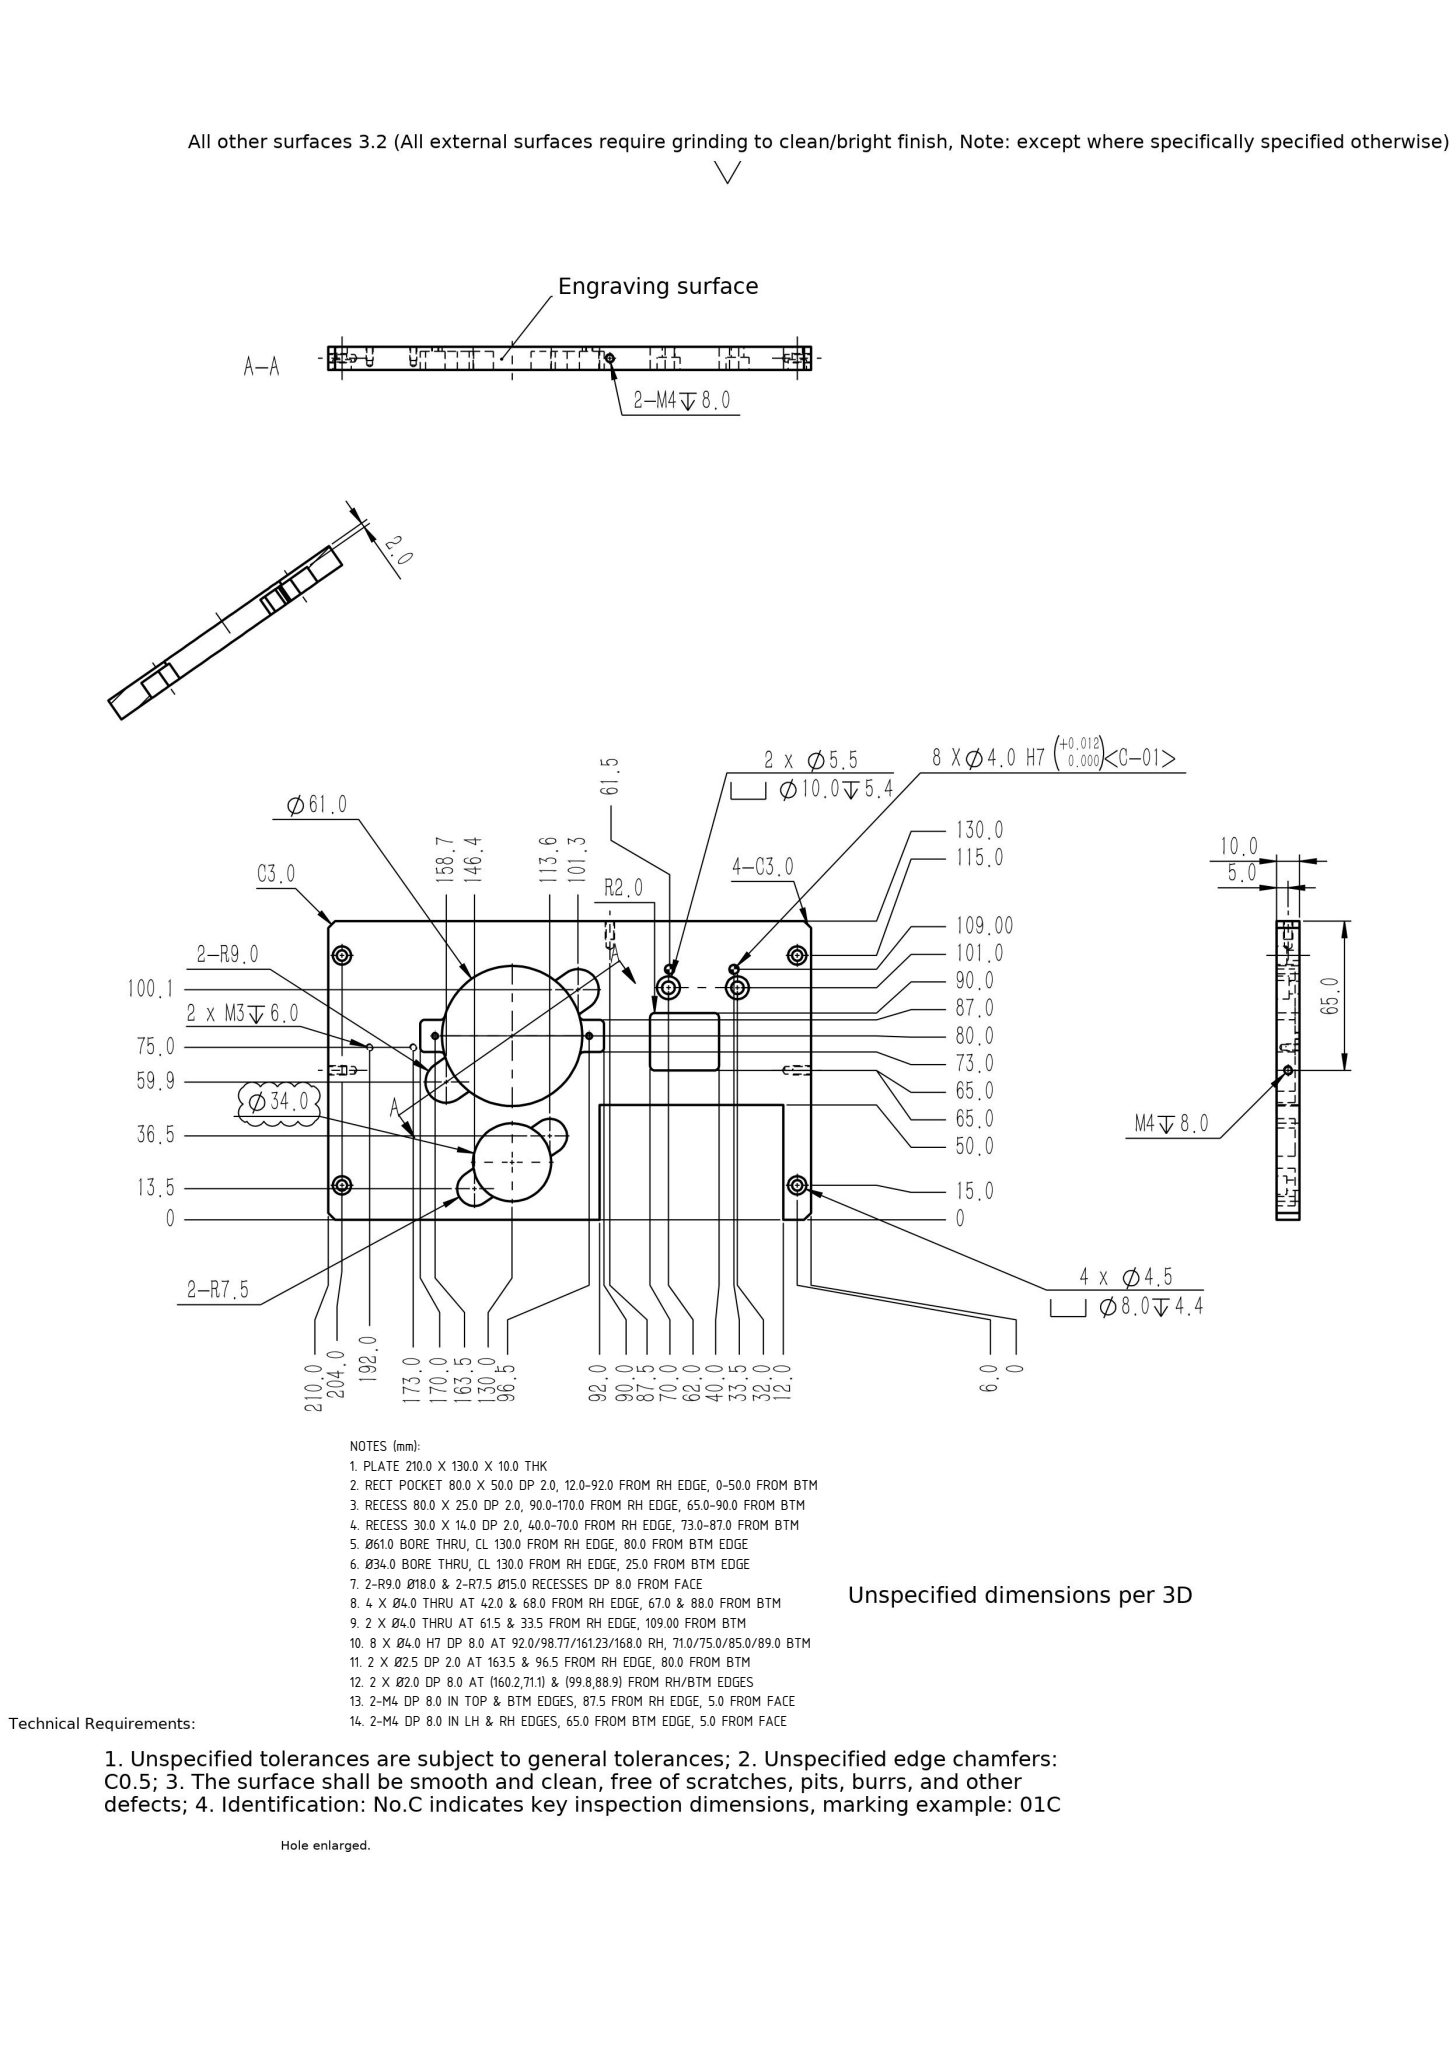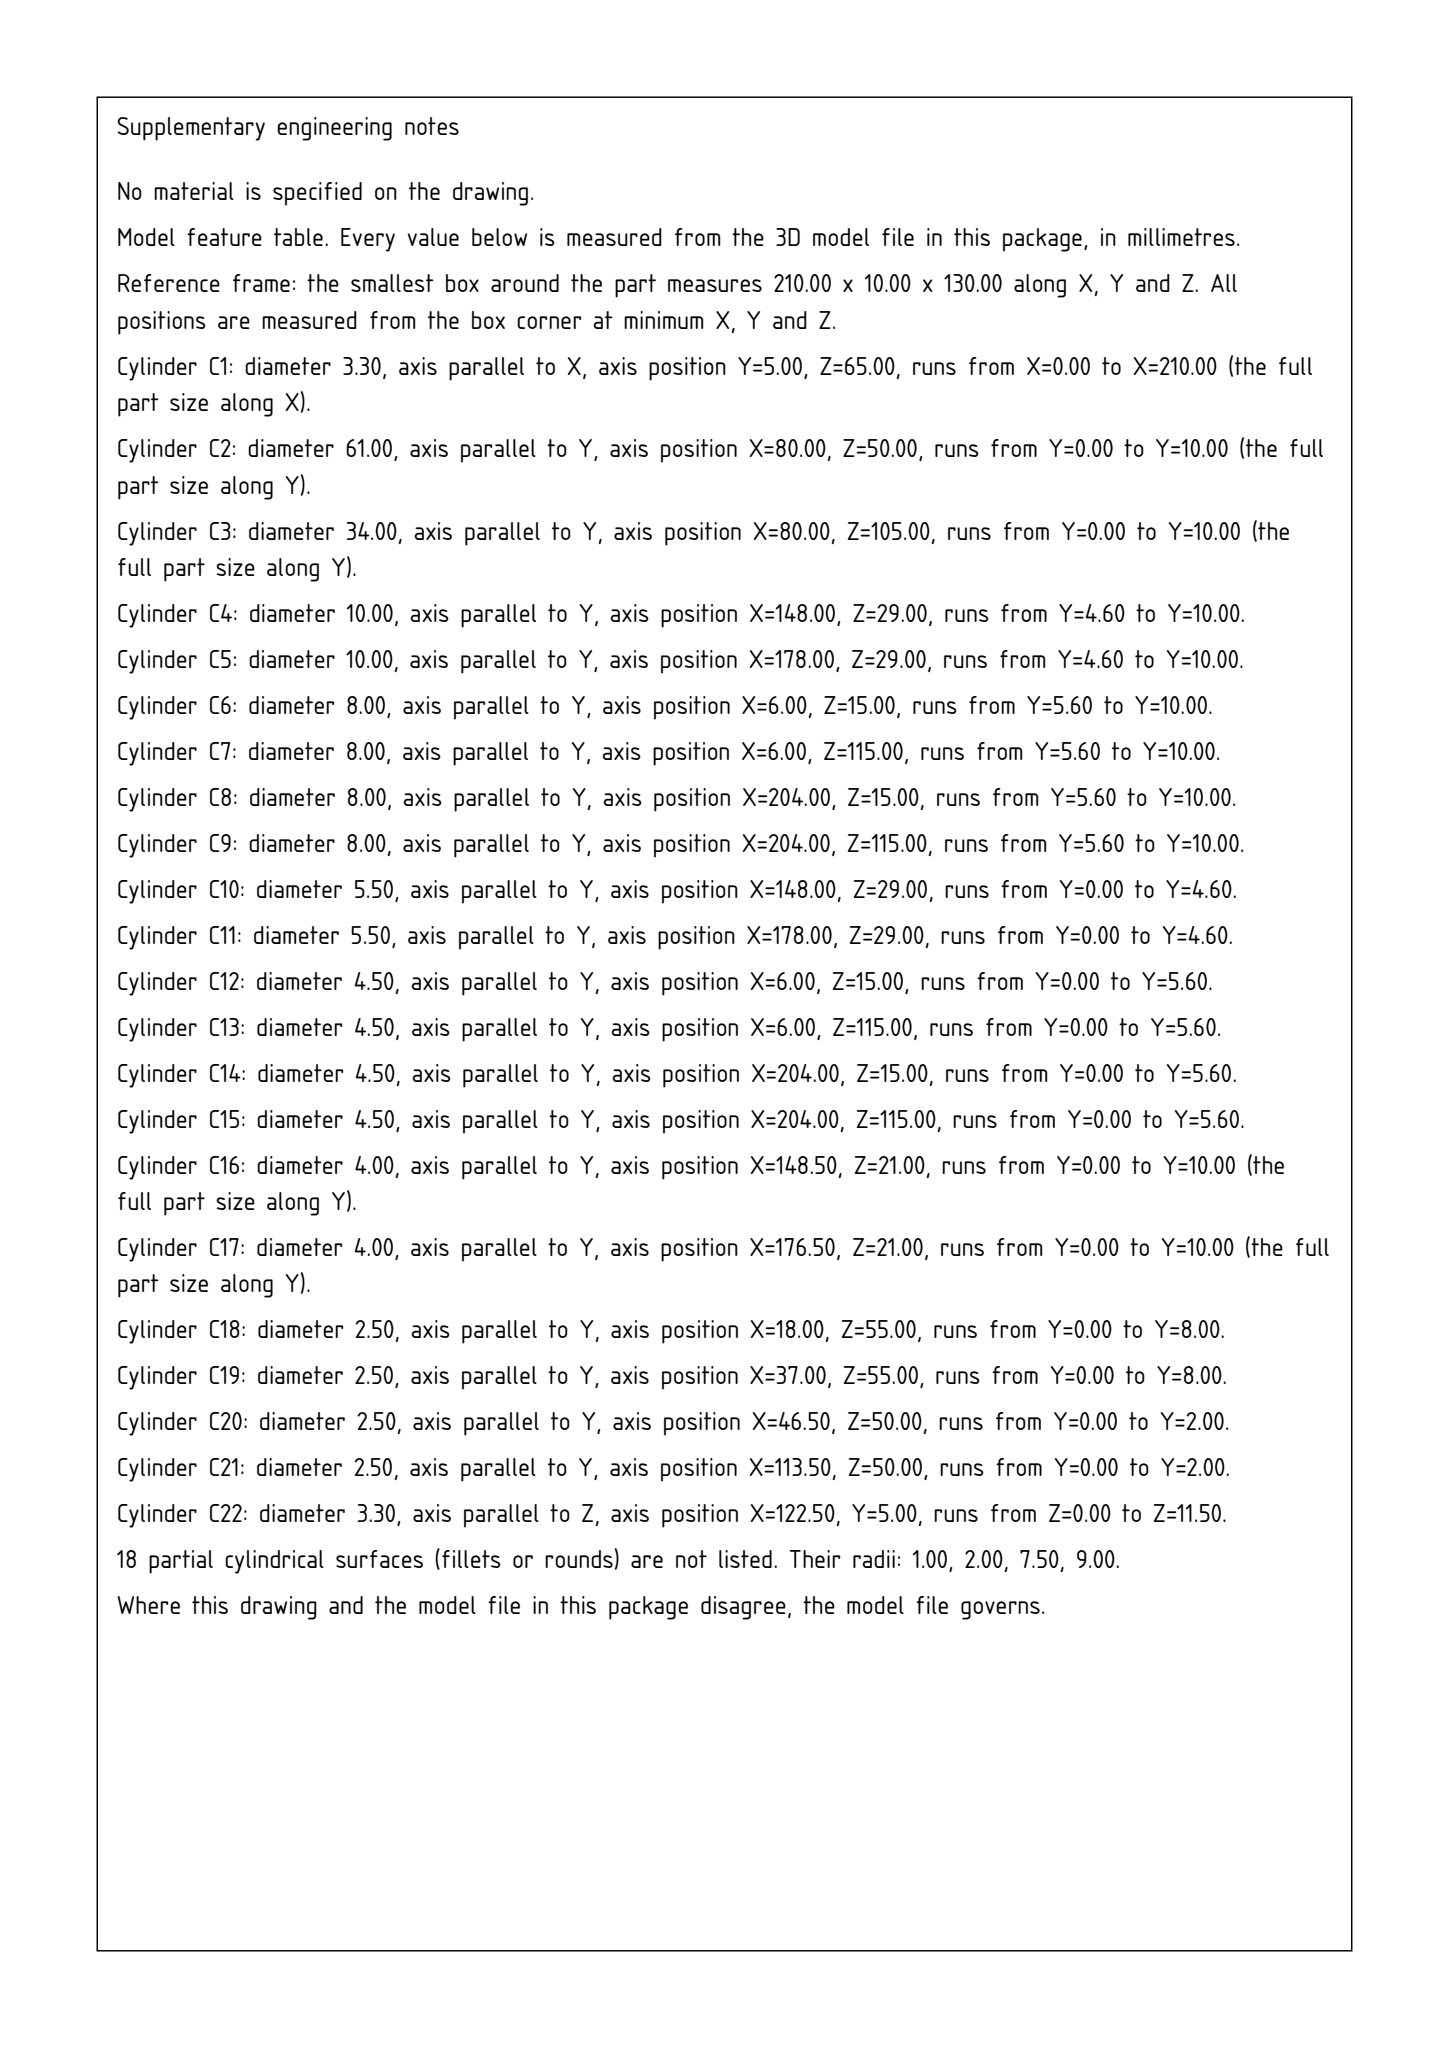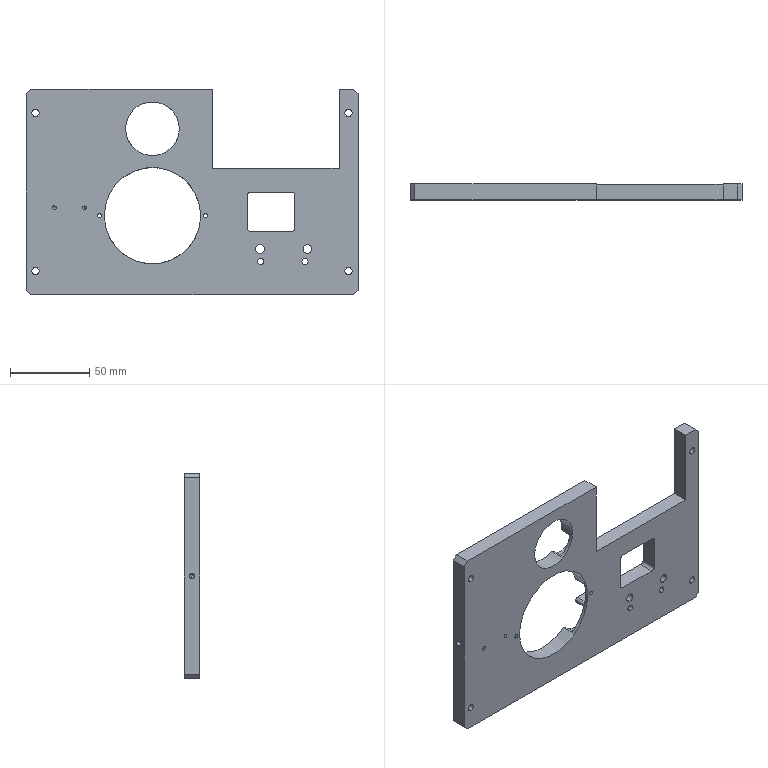Part | SolidWorks | mm | 1 solid | 121 faces | box 210 x 10 x 130 mm | volume 176179 mm3 | cylinder 67 | plane 44 | cone 10 | commonest cylinder face diameters 4 x16 2.5 x8 8 x8 4.5 x8 3.3 x6 10 x4 5.5 x4 2 x3
Drawing notes:
PLATE 210.0 X 130.0 X 10.0 THK | from the solid: bbox_xyz 210.0 x 130.0 x 10.0 (plate thk = y 10.0)
RECT POCKET 80.0 X 50.0 DP 2.0, 12.0-92.0 FROM RH EDGE, 0-50.0 FROM BTM | from the solid: x planes 118.0/198.0 & z planes 80.0/130.0; floor plane y=2.0
RECESS 80.0 X 25.0 DP 2.0, 90.0-170.0 FROM RH EDGE, 65.0-90.0 FROM BTM | from the solid: x planes 40.0/120.0 & z planes 40.0/65.0; floor plane y=2.0
RECESS 30.0 X 14.0 DP 2.0, 40.0-70.0 FROM RH EDGE, 73.0-87.0 FROM BTM | from the solid: x planes 140.0/170.0 & z planes 43.0/57.0; floor y=2.0
Ø61.0 BORE THRU, CL 130.0 FROM RH EDGE, 80.0 FROM BTM EDGE | from the solid: cyl dia 61.0 axis y at x=80.0,z=50.0, length 10.0 = plate thk
Ø34.0 BORE THRU, CL 130.0 FROM RH EDGE, 25.0 FROM BTM EDGE | from the solid: cyl dia 34.0 axis y at x=80.0,z=105.0, length 10.0 = plate thk
2-R9.0 Ø18.0 & 2-R7.5 Ø15.0 RECESSES DP 8.0 FROM FACE | from the solid: dia 18.0 at (51.33,70.08)/(108.67,29.92), dia 15.0 at (63.62,116.47)/(96.38,93.53), L=8.0
4 X Ø4.0 THRU AT 42.0 & 68.0 FROM RH EDGE, 67.0 & 88.0 FROM BTM | from the solid: dia 4.0 axis y at x=142.0/168.0, z=42.0/63.0, length 10.0 = thru
2 X Ø4.0 THRU AT 61.5 & 33.5 FROM RH EDGE, 109.00 FROM BTM | from the solid: dia 4.0 axis y at (148.5,21.0) & (176.5,21.0), length 10.0 = thru
8 X Ø4.0 H7 DP 8.0 AT 92.0/98.77/161.23/168.0 RH, 71.0/75.0/85.0/89.0 BTM | from the solid: 8 blind cyls dia 4.0 axis y L=8.0 at x=118.0/111.23/48.77/42.0, z=59.0/55.0/45.0/41.0
2 X Ø2.5 DP 2.0 AT 163.5 & 96.5 FROM RH EDGE, 80.0 FROM BTM | from the solid: dia 2.5 axis y at (46.5,50.0) & (113.5,50.0), length 2.0
2 X Ø2.0 DP 8.0 AT (160.2,71.1) & (99.8,88.9) FROM RH/BTM EDGES | from the solid: cyl dia 2.0 axis y len 8.0 at (49.8,58.94) and (110.2,41.06) -> 210-x, 130-z
2-M4 DP 8.0 IN TOP & BTM EDGES, 87.5 FROM RH EDGE, 5.0 FROM FACE | from the solid: dia 3.3 tap-drill axis z at x=122.5, y=5.0, len 11.5 -> 210-122.5=87.5
2-M4 DP 8.0 IN LH & RH EDGES, 65.0 FROM BTM EDGE, 5.0 FROM FACE | from the solid: dia 3.3 tap-drill axis x at y=5.0, z=65.0, len 11.5 at x=0 and x=210 ends
build123d program:
from build123d import *

# Parameters (mm, degrees)
SKETCH1_W                                       = 390
SKETCH1_H                                       = 182
BOSS_EXTRUDE1_DEPTH                             = 130
SHELL1_T                                        = -10
SKETCH7_W                                       = 60
SKETCH7_H                                       = 80
CUT_EXTRUDE4_DEPTH                              = 10
SKETCH8_W                                       = 404.233
SKETCH8_H                                       = 242.582
CUT_EXTRUDE5_DEPTH                              = 559.5
SKETCH46_W                                      = 210
SKETCH46_H                                      = 130
CUT_EXTRUDE13_DEPTH                             = 10
M4_HEX_SOCKET_HEAD_CAP_SCREW_CBORE2_D           = 4.5
M4_HEX_SOCKET_HEAD_CAP_SCREW_CBORE2_CBORE_D     = 8
M4_HEX_SOCKET_HEAD_CAP_SCREW_CBORE2_CBORE_DEPTH = 4.4
SKETCH67_W                                      = 30
SKETCH67_H                                      = 130
BOSS_EXTRUDE2_DEPTH                             = 10
SKETCH68_R                                      = 17
CUT_EXTRUDE14_DEPTH                             = 178.2
LPATTERN1_COUNT                                 = 2
LPATTERN1_PITCH                                 = 198
M4_TAPPED_HOLE1_D                               = 3.3
M4_TAPPED_HOLE1_DEPTH                           = 11.5
M4_TAPPED_HOLE1_TIP                             = 0.9914
M4_TAPPED_HOLE2_D                               = 3.3
M4_TAPPED_HOLE2_DEPTH                           = 11.5
M4_TAPPED_HOLE2_TIP                             = 0.9914
M4_TAPPED_HOLE3_D                               = 3.3
M4_TAPPED_HOLE3_DEPTH                           = 11.5
M4_TAPPED_HOLE3_TIP                             = 0.9914
CHAMFER1_SIZE                                   = 3
SKETCH78_R                                      = 30.5
CUT_EXTRUDE15_DEPTH                             = 10
SKETCH90_W                                      = 30
SKETCH90_H                                      = 25
CUT_EXTRUDE21_DEPTH                             = 10
M5_HEX_SOCKET_HEAD_CAP_SCREW_CBORE3_D           = 5.5
M5_HEX_SOCKET_HEAD_CAP_SCREW_CBORE3_CBORE_D     = 10
M5_HEX_SOCKET_HEAD_CAP_SCREW_CBORE3_CBORE_DEPTH = 5.4
F_4_0_4_DIAMETER_HOLE2_D                        = 4
SKETCH95_W                                      = 80
SKETCH95_H                                      = 14
CUT_EXTRUDE22_DEPTH                             = 8
FILLET1_R                                       = 2
M3_TAPPED_HOLE1_D                               = 2.5
FILLET3_R                                       = 2
CUT_EXTRUDE24_DEPTH                             = 8
CUT_EXTRUDE25_DEPTH                             = 8
FILLET4_R                                       = 1
M3_TAPPED_HOLE2_D                               = 2.5
M3_TAPPED_HOLE2_DEPTH                           = 8
M3_TAPPED_HOLE2_TIP                             = 0.7511
SKETCH103_W                                     = 80
SKETCH103_H                                     = 50
CUT_EXTRUDE26_DEPTH                             = 10


with BuildPart() as part:
    # Sketch1 → Boss-Extrude1 (new body)
    with BuildSketch(Plane.XY):
        with Locations((135, -56)):
            Rectangle(SKETCH1_W, SKETCH1_H)
    extrude(amount=BOSS_EXTRUDE1_DEPTH)

    # Shell1
    shell1_openings = [part.faces().sort_by_distance(p)[0] for p in [
        (135, -56, 0),
        (135, -147, 65),
    ]]
    offset(amount=SHELL1_T, openings=shell1_openings, kind=Kind.INTERSECTION)

    # Sketch7 → Cut-Extrude4 (cut)
    with BuildSketch(Plane(origin=(330, 0, 0), x_dir=(0, 0, -1), z_dir=(1, 0, 0))):
        with Locations((-30, -75)):
            Rectangle(SKETCH7_W, SKETCH7_H)
    extrude(amount=-CUT_EXTRUDE4_DEPTH, mode=Mode.SUBTRACT)

    # Sketch8 → Cut-Extrude5 (cut, symmetric)
    with BuildSketch(Plane(origin=(330, 0, 0), x_dir=(0, 0, -1), z_dir=(1, 0, 0))):
        with Locations((-49.9, -96.291)):
            Rectangle(SKETCH8_W, SKETCH8_H)
    extrude(amount=CUT_EXTRUDE5_DEPTH, both=True, mode=Mode.SUBTRACT)

    # Sketch46 → Cut-Extrude13 (cut)
    with BuildSketch(Plane(origin=(0, 35, 0), x_dir=(1, 0, 0), z_dir=(0, 1, 0))):
        with Locations((225, -65)):
            Rectangle(SKETCH46_W, SKETCH46_H)
    extrude(amount=-CUT_EXTRUDE13_DEPTH, mode=Mode.SUBTRACT)

    # M4 Hex Socket Head Cap Screw CBORE2 (through all)
    with Locations(Plane(origin=(0, 35, 0), x_dir=(1, 0, 0), z_dir=(0, 1, 0))):
        with Locations((114, -15), (114, -115)):
            m4_hex_socket_head_cap_screw_cbore2 = CounterBoreHole(M4_HEX_SOCKET_HEAD_CAP_SCREW_CBORE2_D / 2, M4_HEX_SOCKET_HEAD_CAP_SCREW_CBORE2_CBORE_D / 2, M4_HEX_SOCKET_HEAD_CAP_SCREW_CBORE2_CBORE_DEPTH)

    # Sketch67 → Boss-Extrude2 (add)
    with BuildSketch(Plane(origin=(0, 35, 0), x_dir=(1, 0, 0), z_dir=(0, 1, 0))):
        with Locations((-75, -65)):
            Rectangle(SKETCH67_W, SKETCH67_H)
    extrude(amount=-BOSS_EXTRUDE2_DEPTH)

    # Sketch68 → Cut-Extrude14 (cut, through all)
    with BuildSketch(Plane(origin=(0, 35, 0), x_dir=(1, 0, 0), z_dir=(0, 1, 0))):
        with Locations(Location((-10, -105, 0), (0, 0, 180))):
            Circle(SKETCH68_R)
    extrude(amount=-CUT_EXTRUDE14_DEPTH, mode=Mode.SUBTRACT)

    # LPattern1: M4 Hex Socket Head Cap Screw CBORE2 ×2
    with Locations(*[(-i * LPATTERN1_PITCH, 0, 0) for i in range(1, LPATTERN1_COUNT)]):
        add(m4_hex_socket_head_cap_screw_cbore2, mode=Mode.SUBTRACT)

    # M4 Tapped Hole1
    with Locations(Plane(origin=(0, 0, 0), x_dir=(-1, 0, 0), z_dir=(0, 0, -1))):
        with Locations((-32.5, 30)):
            Hole(M4_TAPPED_HOLE1_D / 2, depth=M4_TAPPED_HOLE1_DEPTH)
            with Locations((0, 0, -(M4_TAPPED_HOLE1_DEPTH + M4_TAPPED_HOLE1_TIP / 2))):  # 118° drill point
                Cone(0, M4_TAPPED_HOLE1_D / 2, M4_TAPPED_HOLE1_TIP, mode=Mode.SUBTRACT)

    # M4 Tapped Hole2
    with Locations(Plane.ZY.offset(90)):
        with Locations((65, 30)):
            Hole(M4_TAPPED_HOLE2_D / 2, depth=M4_TAPPED_HOLE2_DEPTH)
            with Locations((0, 0, -(M4_TAPPED_HOLE2_DEPTH + M4_TAPPED_HOLE2_TIP / 2))):  # 118° drill point
                Cone(0, M4_TAPPED_HOLE2_D / 2, M4_TAPPED_HOLE2_TIP, mode=Mode.SUBTRACT)

    # M4 Tapped Hole3
    with Locations(Plane(origin=(120, 0, 0), x_dir=(0, 0, -1), z_dir=(1, 0, 0))):
        with Locations((-65, 30)):
            Hole(M4_TAPPED_HOLE3_D / 2, depth=M4_TAPPED_HOLE3_DEPTH)
            with Locations((0, 0, -(M4_TAPPED_HOLE3_DEPTH + M4_TAPPED_HOLE3_TIP / 2))):  # 118° drill point
                Cone(0, M4_TAPPED_HOLE3_D / 2, M4_TAPPED_HOLE3_TIP, mode=Mode.SUBTRACT)

    # Chamfer1
    chamfer1_edges = [part.edges().sort_by_distance(p)[0] for p in [
        (120, 30, 130),
        (120, 30, 0),
        (-90, 30, 130),
        (-90, 30, 0),
    ]]
    chamfer(chamfer1_edges, length=CHAMFER1_SIZE)

    # Sketch78 → Cut-Extrude15 (cut)
    with BuildSketch(Plane(origin=(0, 35, 0), x_dir=(1, 0, 0), z_dir=(0, 1, 0))):
        with Locations(Location((-10, -50, 0), (0, 0, 180))):
            Circle(SKETCH78_R)
    extrude(amount=-CUT_EXTRUDE15_DEPTH, mode=Mode.SUBTRACT)

    # Sketch90 → Cut-Extrude21 (cut)
    with BuildSketch(Plane(origin=(0, 35, 0), x_dir=(1, 0, 0), z_dir=(0, 1, 0))):
        with Locations((65, -52.5)):
            Rectangle(SKETCH90_W, SKETCH90_H)
    extrude(amount=-CUT_EXTRUDE21_DEPTH, mode=Mode.SUBTRACT)

    # M5 Hex Socket Head Cap Screw CBORE3 (through all)
    with Locations(Plane(origin=(0, 35, 0), x_dir=(1, 0, 0), z_dir=(0, 1, 0))):
        with Locations((88, -29), (58, -29)):
            CounterBoreHole(M5_HEX_SOCKET_HEAD_CAP_SCREW_CBORE3_D / 2, M5_HEX_SOCKET_HEAD_CAP_SCREW_CBORE3_CBORE_D / 2, M5_HEX_SOCKET_HEAD_CAP_SCREW_CBORE3_CBORE_DEPTH)

    # 4.0 _4_ Diameter Hole2 (through all)
    with Locations(Plane(origin=(0, 35, 0), x_dir=(1, 0, 0), z_dir=(0, 1, 0))):
        with Locations((86.5, -21), (58.5, -21)):
            Hole(F_4_0_4_DIAMETER_HOLE2_D / 2)

    # Sketch95 → Cut-Extrude22 (cut)
    with BuildSketch(Plane(origin=(0, 35, 0), x_dir=(1, 0, 0), z_dir=(0, 1, 0))):
        with Locations((-10, -50)):
            Rectangle(SKETCH95_W, SKETCH95_H)
    extrude(amount=-CUT_EXTRUDE22_DEPTH, mode=Mode.SUBTRACT)

    # Fillet1
    fillet1_edges = [part.edges().sort_by_distance(p)[0] for p in [
        (19.686, 31, 57),
        (19.686, 31, 43),
        (-39.686, 31, 57),
        (-39.686, 31, 43),
        (-50, 31, 43),
        (30, 31, 57),
        (-50, 31, 57),
        (30, 31, 43),
    ]]
    fillet(fillet1_edges, radius=FILLET1_R)

    # M3 Tapped Hole1 (through all)
    with Locations(Plane(origin=(0, 27, 0), x_dir=(1, 0, 0), z_dir=(0, 1, 0))):
        with Locations((-43.5, -50), (23.5, -50)):
            Hole(M3_TAPPED_HOLE1_D / 2)

    # Fillet3
    fillet3_edges = [part.edges().sort_by_distance(p)[0] for p in [
        (80, 30, 40),
        (80, 30, 65),
        (50, 30, 65),
        (50, 30, 40),
    ]]
    fillet(fillet3_edges, radius=FILLET3_R)

    # Sketch99 → Cut-Extrude24 (cut)
    with BuildSketch(Plane(origin=(0, 35, 0), x_dir=(1, 0, 0), z_dir=(0, 1, 0))):
        with BuildLine():
            Line((23.833, -37.297), (-33.508, -77.448))
            ThreePointArc((-33.508, -77.448), (-46.043, -75.237), (-43.833, -62.703))
            Line((-43.833, -62.703), (13.508, -22.552))
            ThreePointArc((13.508, -22.552), (26.043, -24.763), (23.833, -37.297))
        make_face()
    extrude(amount=-CUT_EXTRUDE24_DEPTH, mode=Mode.SUBTRACT)

    # Sketch100 → Cut-Extrude25 (cut)
    with BuildSketch(Plane(origin=(0, 35, 0), x_dir=(1, 0, 0), z_dir=(0, 1, 0))):
        with BuildLine():
            Line((10.685, -99.672), (-22.081, -122.615))
            ThreePointArc((-22.081, -122.615), (-32.527, -120.773), (-30.685, -110.328))
            Line((-30.685, -110.328), (2.081, -87.385))
            ThreePointArc((2.081, -87.385), (12.527, -89.227), (10.685, -99.672))
        make_face()
    extrude(amount=-CUT_EXTRUDE25_DEPTH, mode=Mode.SUBTRACT)

    # Fillet4
    fillet4_edges = [part.edges().sort_by_distance(p)[0] for p in [
        (-39.034, 31, 59.343),
        (19.034, 31, 40.657),
    ]]
    fillet(fillet4_edges, radius=FILLET4_R)

    # M3 Tapped Hole2
    with Locations(Plane(origin=(0, 25, 0), x_dir=(-1, 0, 0), z_dir=(0, -1, 0))):
        with Locations((53, -55), (72, -55)):
            Hole(M3_TAPPED_HOLE2_D / 2, depth=M3_TAPPED_HOLE2_DEPTH)
            with Locations((0, 0, -(M3_TAPPED_HOLE2_DEPTH + M3_TAPPED_HOLE2_TIP / 2))):  # 118° drill point
                Cone(0, M3_TAPPED_HOLE2_D / 2, M3_TAPPED_HOLE2_TIP, mode=Mode.SUBTRACT)

    # Sketch103 → Cut-Extrude26 (cut)
    with BuildSketch(Plane(origin=(0, 35, 0), x_dir=(1, 0, 0), z_dir=(0, 1, 0))):
        with Locations((68, -105)):
            Rectangle(SKETCH103_W, SKETCH103_H)
    extrude(amount=-CUT_EXTRUDE26_DEPTH, mode=Mode.SUBTRACT)


solid = part.part